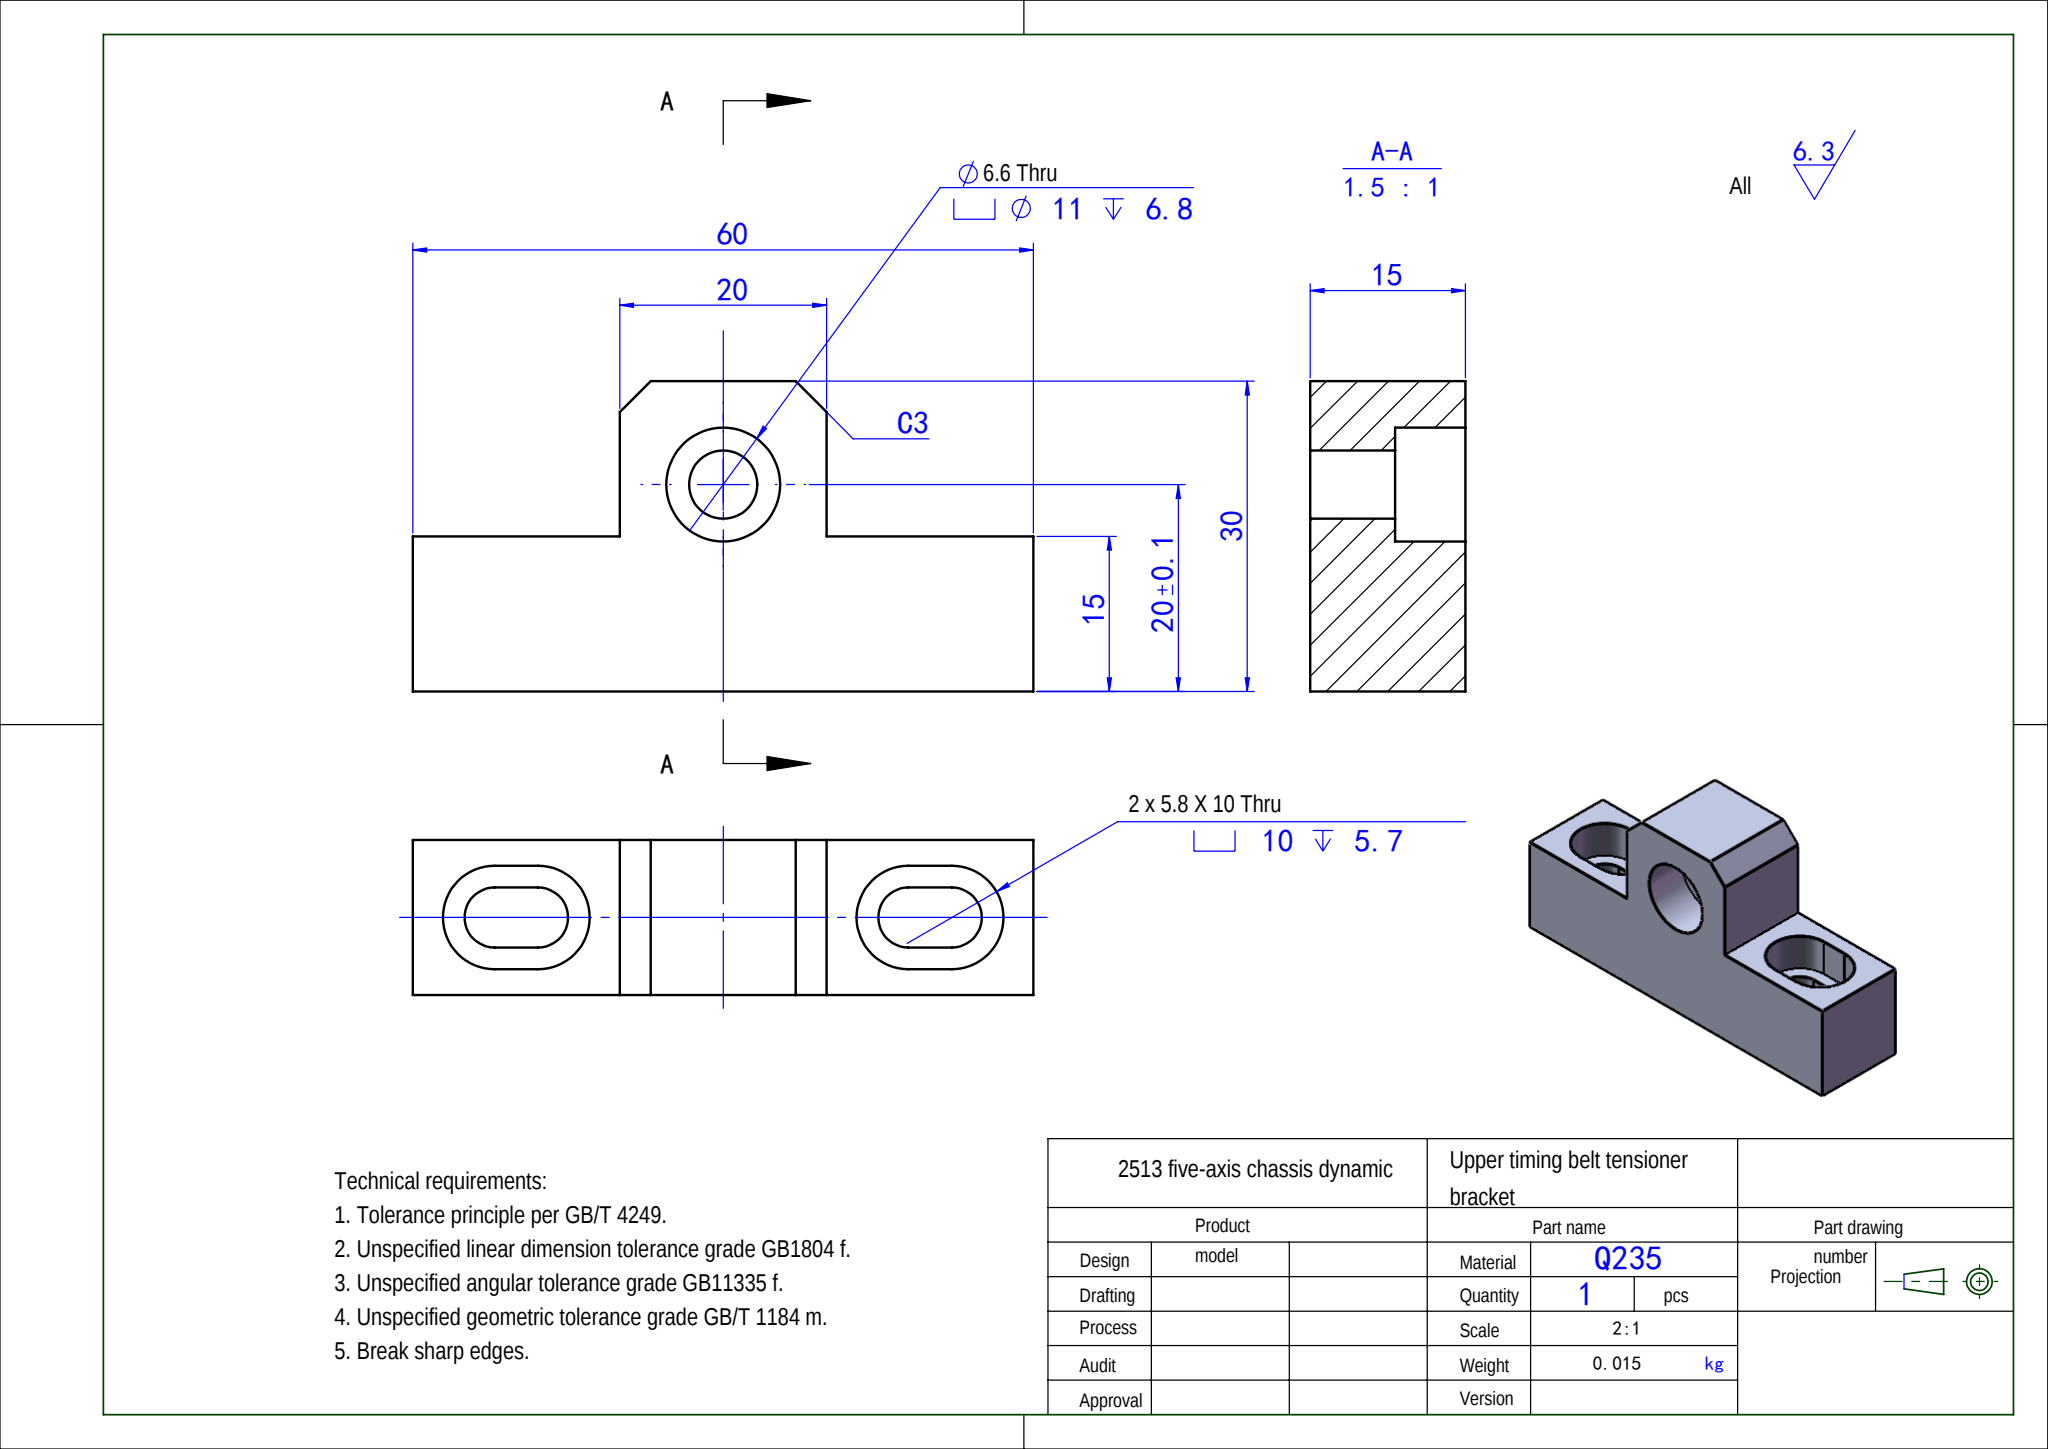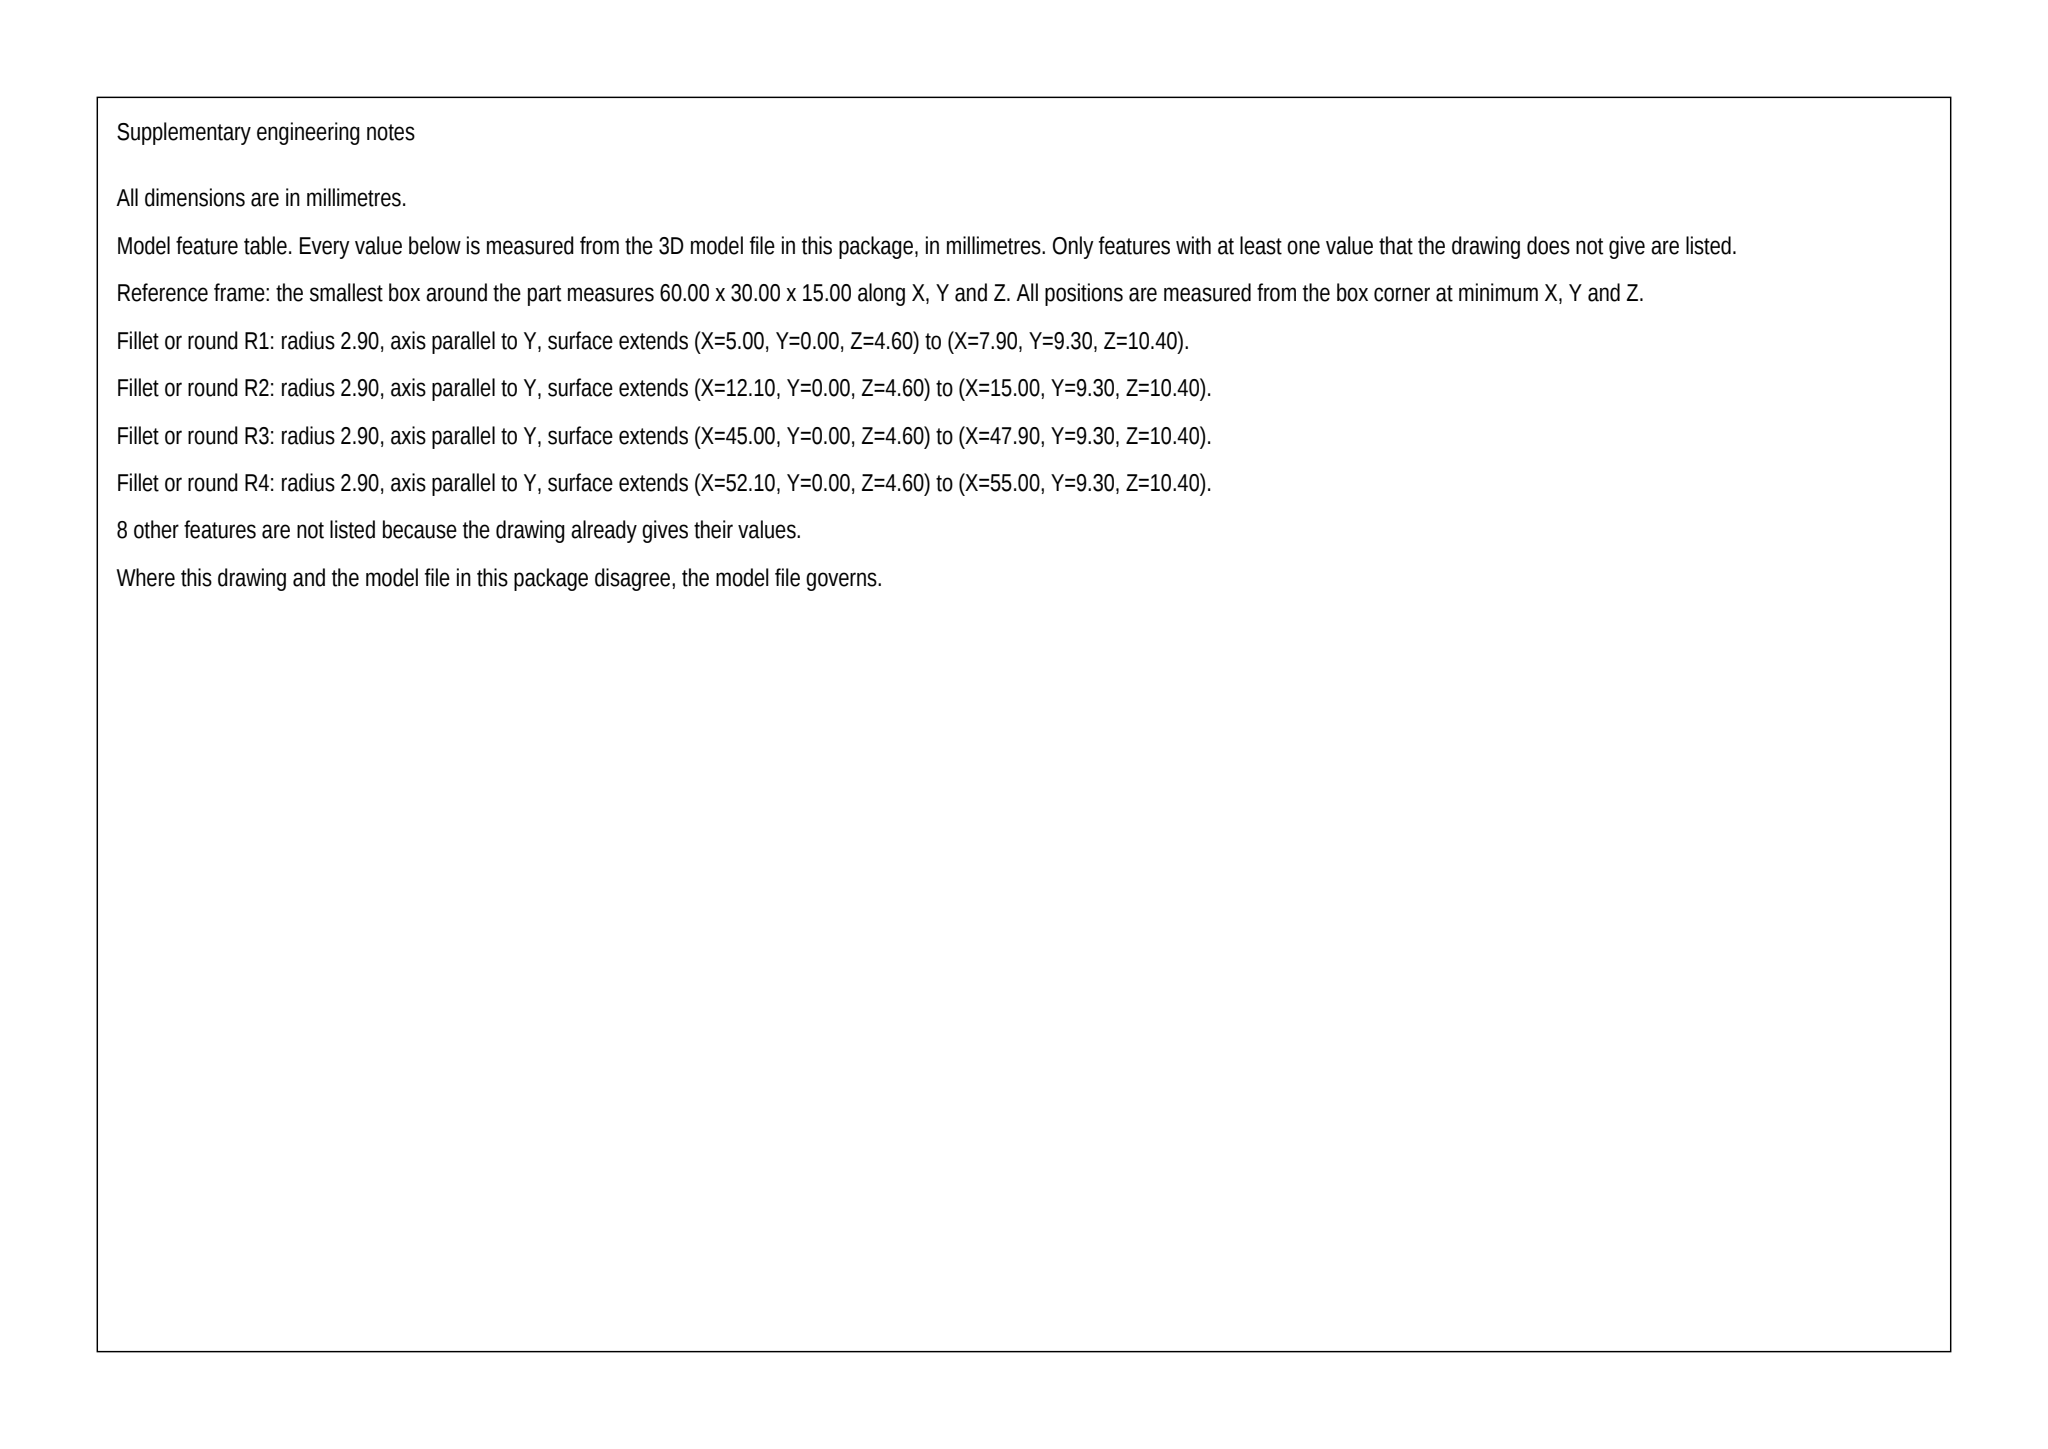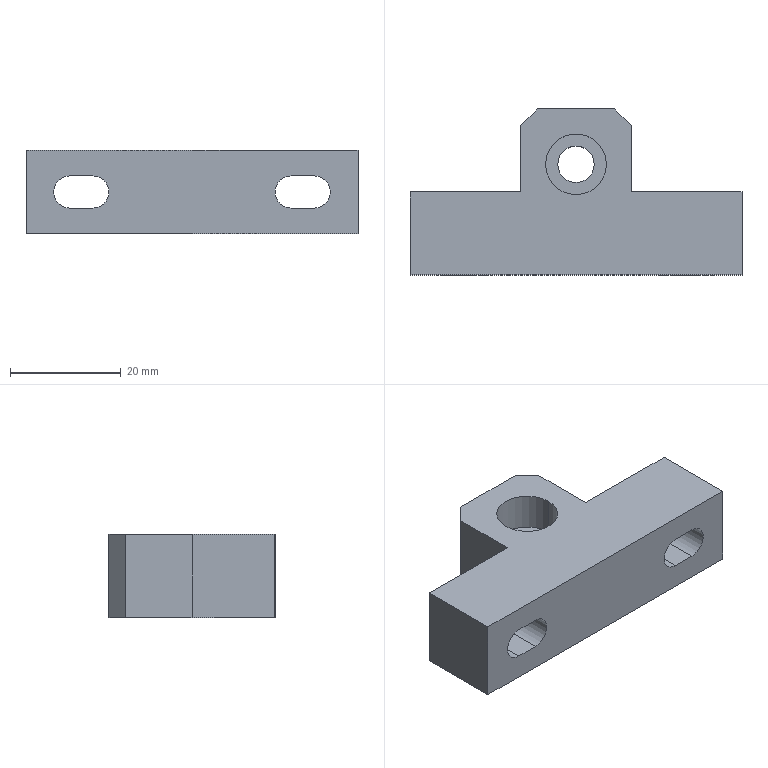Part | SolidWorks | mm | material Q235 | 1 solid | 35 faces | box 60 x 30 x 15 mm | volume 14620 mm3 | plane 23 | cylinder 12 | commonest cylinder face diameters 5.8 x4 10 x4 11 x2 6.6 x2